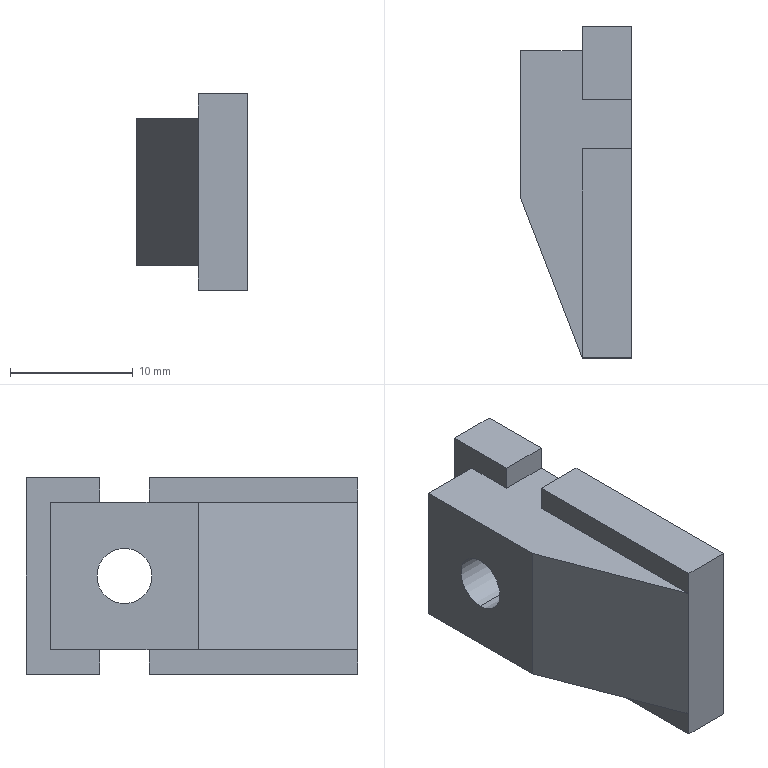Component | SolidWorks | ClampingBlock-2 | 1 solid | 24 faces | box 9 x 27 x 16 mm | volume 2480 mm3 | plane 20 | cylinder 4 | commonest cylinder face diameters 8 x2 4.5 x2
build123d program:
from build123d import *

# Parameters (mm, degrees)
BOSS_EXTRUDE1_DEPTH                             = 8
M4_HEX_SOCKET_HEAD_CAP_SCREW_CBORE2_D           = 4.5
M4_HEX_SOCKET_HEAD_CAP_SCREW_CBORE2_DEPTH       = 10.1
M4_HEX_SOCKET_HEAD_CAP_SCREW_CBORE2_CBORE_D     = 8
M4_HEX_SOCKET_HEAD_CAP_SCREW_CBORE2_CBORE_DEPTH = 4.4
M4_HEX_SOCKET_HEAD_CAP_SCREW_CBORE2_TIP         = 1.352
SKETCH4_W                                       = 5
SKETCH4_H                                       = 2
CUT_EXTRUDE1_DEPTH                              = 28.749
SKETCH5_W                                       = 2
SKETCH5_H                                       = 4
CUT_EXTRUDE2_DEPTH                              = 16


with BuildPart() as part:
    # Sketch1 → Boss-Extrude1 (new, symmetric)
    with BuildSketch(Plane.XY):
        Polygon((0, 0), (0, 27), (4, 27), (4, 25), (9, 25), (9, 13), (4, 0), align=None)
    extrude(amount=BOSS_EXTRUDE1_DEPTH, both=True)

    # M4 Hex Socket Head Cap Screw CBORE2
    with Locations(Plane(origin=(0, 19, 0), x_dir=(0, 0, -1), z_dir=(-1, 0, 0))):
        with Locations((0, 0)):
            CounterBoreHole(M4_HEX_SOCKET_HEAD_CAP_SCREW_CBORE2_D / 2, M4_HEX_SOCKET_HEAD_CAP_SCREW_CBORE2_CBORE_D / 2, M4_HEX_SOCKET_HEAD_CAP_SCREW_CBORE2_CBORE_DEPTH, depth=M4_HEX_SOCKET_HEAD_CAP_SCREW_CBORE2_DEPTH)
            with Locations((0, 0, -(M4_HEX_SOCKET_HEAD_CAP_SCREW_CBORE2_DEPTH + M4_HEX_SOCKET_HEAD_CAP_SCREW_CBORE2_TIP / 2))):  # 118° drill point
                Cone(0, M4_HEX_SOCKET_HEAD_CAP_SCREW_CBORE2_D / 2, M4_HEX_SOCKET_HEAD_CAP_SCREW_CBORE2_TIP, mode=Mode.SUBTRACT)

    # Sketch4 → Cut-Extrude1 (cut, through all)
    with BuildSketch(Plane(origin=(0, 25, 0), x_dir=(1, 0, 0), z_dir=(0, 1, 0))):
        with Locations((6.5, 7)):
            Rectangle(SKETCH4_W, SKETCH4_H)
        with Locations((6.5, -7)):
            Rectangle(SKETCH4_W, SKETCH4_H)
    extrude(amount=-CUT_EXTRUDE1_DEPTH, mode=Mode.SUBTRACT)

    # Sketch5 → Cut-Extrude2 (cut)
    with BuildSketch(Plane(origin=(4, 0, 0), x_dir=(0, 0, -1), z_dir=(1, 0, 0))):
        with Locations((-7, 19)):
            Rectangle(SKETCH5_W, SKETCH5_H)
        with Locations((7, 19)):
            Rectangle(SKETCH5_W, SKETCH5_H)
    extrude(amount=-CUT_EXTRUDE2_DEPTH, mode=Mode.SUBTRACT)


solid = part.part

# Placed as in the assembly
solid = solid.moved(Location((38.658, -220.962, 175.844), (-180, 0, 180)))
STEP:
#1=COLOUR_RGB('',0.7922,0.8196,0.9333);
#2=FILL_AREA_STYLE_COLOUR('',#1);
#3=FILL_AREA_STYLE('',(#2));
#4=SURFACE_STYLE_FILL_AREA(#3);
#5=SURFACE_SIDE_STYLE('',(#4));
#6=SURFACE_STYLE_USAGE(.BOTH.,#5);
#7=PRESENTATION_STYLE_ASSIGNMENT((#6));
#8=CARTESIAN_POINT('',(1.349,-7.951,7.08));
#9=VERTEX_POINT('',#8);
#10=CARTESIAN_POINT('',(1.349,-7.951,6.766));
#11=VERTEX_POINT('',#10);
#12=CARTESIAN_POINT('',(1.349,-7.951,6.923));
#13=DIRECTION('',(1.,-0.,0.));
#14=DIRECTION('',(0.,0.,-1.));
#15=AXIS2_PLACEMENT_3D('',#12,#13,#14);
#16=CIRCLE('',#15,0.1575);
#17=EDGE_CURVE('',#9,#11,#16,.T.);
#18=ORIENTED_EDGE('',*,*,#17,.F.);
#19=CARTESIAN_POINT('',(1.522,-7.951,7.08));
#20=VERTEX_POINT('',#19);
#21=CARTESIAN_POINT('',(1.522,-7.951,7.08));
#22=DIRECTION('',(1.,-0.,0.));
#23=VECTOR('',#22,39.37);
#24=LINE('',#21,#23);
#25=EDGE_CURVE('',#9,#20,#24,.T.);
#26=ORIENTED_EDGE('',*,*,#25,.T.);
#27=CARTESIAN_POINT('',(1.522,-7.951,6.766));
#28=VERTEX_POINT('',#27);
#29=CARTESIAN_POINT('',(1.522,-7.951,6.923));
#30=DIRECTION('',(1.,-0.,0.));
#31=DIRECTION('',(0.,0.,-1.));
#32=AXIS2_PLACEMENT_3D('',#29,#30,#31);
#33=CIRCLE('',#32,0.1575);
#34=EDGE_CURVE('',#20,#28,#33,.T.);
#35=ORIENTED_EDGE('',*,*,#34,.T.);
#36=CARTESIAN_POINT('',(1.522,-7.951,6.766));
#37=DIRECTION('',(1.,-0.,0.));
#38=VECTOR('',#37,39.37);
#39=LINE('',#36,#38);
#40=EDGE_CURVE('',#11,#28,#39,.T.);
#41=ORIENTED_EDGE('',*,*,#40,.F.);
#42=EDGE_LOOP('',(#18,#26,#35,#41));
#43=FACE_OUTER_BOUND('',#42,.T.);
#44=CARTESIAN_POINT('',(1.522,-7.951,6.923));
#45=DIRECTION('',(1.,-0.,0.));
#46=DIRECTION('',(0.,0.,-1.));
#47=AXIS2_PLACEMENT_3D('',#44,#45,#46);
#48=CYLINDRICAL_SURFACE('',#47,0.1575);
#49=ADVANCED_FACE('',(#43),#48,.F.);
#50=CARTESIAN_POINT('',(1.168,-7.951,7.012));
#51=VERTEX_POINT('',#50);
#52=CARTESIAN_POINT('',(1.168,-7.951,6.834));
#53=VERTEX_POINT('',#52);
#54=CARTESIAN_POINT('',(1.168,-7.951,6.923));
#55=DIRECTION('',(1.,-0.,0.));
#56=DIRECTION('',(0.,-1.,0.));
#57=AXIS2_PLACEMENT_3D('',#54,#55,#56);
#58=CIRCLE('',#57,0.08858);
#59=EDGE_CURVE('',#51,#53,#58,.T.);
#60=ORIENTED_EDGE('',*,*,#59,.F.);
#61=CARTESIAN_POINT('',(1.349,-7.951,7.012));
#62=VERTEX_POINT('',#61);
#63=CARTESIAN_POINT('',(1.522,-7.951,7.012));
#64=DIRECTION('',(1.,-0.,0.));
#65=VECTOR('',#64,39.37);
#66=LINE('',#63,#65);
#67=EDGE_CURVE('',#51,#62,#66,.T.);
#68=ORIENTED_EDGE('',*,*,#67,.T.);
#69=CARTESIAN_POINT('',(1.349,-7.951,6.834));
#70=VERTEX_POINT('',#69);
#71=CARTESIAN_POINT('',(1.349,-7.951,6.923));
#72=DIRECTION('',(1.,-0.,0.));
#73=DIRECTION('',(0.,0.,-1.));
#74=AXIS2_PLACEMENT_3D('',#71,#72,#73);
#75=CIRCLE('',#74,0.08858);
#76=EDGE_CURVE('',#62,#70,#75,.T.);
#77=ORIENTED_EDGE('',*,*,#76,.T.);
#78=CARTESIAN_POINT('',(1.522,-7.951,6.834));
#79=DIRECTION('',(1.,-0.,0.));
#80=VECTOR('',#79,39.37);
#81=LINE('',#78,#80);
#82=EDGE_CURVE('',#53,#70,#81,.T.);
#83=ORIENTED_EDGE('',*,*,#82,.F.);
#84=EDGE_LOOP('',(#60,#68,#77,#83));
#85=FACE_OUTER_BOUND('',#84,.T.);
#86=CARTESIAN_POINT('',(1.522,-7.951,6.923));
#87=DIRECTION('',(1.,-0.,0.));
#88=DIRECTION('',(0.,0.,-1.));
#89=AXIS2_PLACEMENT_3D('',#86,#87,#88);
#90=CYLINDRICAL_SURFACE('',#89,0.08858);
#91=ADVANCED_FACE('',(#85),#90,.F.);
#92=CARTESIAN_POINT('',(1.364,-7.873,7.159));
#93=VERTEX_POINT('',#92);
#94=CARTESIAN_POINT('',(1.364,-7.715,7.159));
#95=VERTEX_POINT('',#94);
#96=CARTESIAN_POINT('',(1.364,-8.699,7.159));
#97=DIRECTION('',(0.,1.,0.));
#98=VECTOR('',#97,39.37);
#99=LINE('',#96,#98);
#100=EDGE_CURVE('',#93,#95,#99,.T.);
#101=ORIENTED_EDGE('',*,*,#100,.F.);
#102=CARTESIAN_POINT('',(1.364,-7.873,7.238));
#103=VERTEX_POINT('',#102);
#104=CARTESIAN_POINT('',(1.364,-7.873,7.159));
#105=DIRECTION('',(0.,-0.,-1.));
#106=VECTOR('',#105,39.37);
#107=LINE('',#104,#106);
#108=EDGE_CURVE('',#103,#93,#107,.T.);
#109=ORIENTED_EDGE('',*,*,#108,.F.);
#110=CARTESIAN_POINT('',(1.364,-7.636,7.238));
#111=VERTEX_POINT('',#110);
#112=CARTESIAN_POINT('',(1.364,-7.636,7.238));
#113=DIRECTION('',(0.,1.,0.));
#114=VECTOR('',#113,39.37);
#115=LINE('',#112,#114);
#116=EDGE_CURVE('',#103,#111,#115,.T.);
#117=ORIENTED_EDGE('',*,*,#116,.T.);
#118=CARTESIAN_POINT('',(1.364,-7.636,6.608));
#119=VERTEX_POINT('',#118);
#120=CARTESIAN_POINT('',(1.364,-7.636,6.608));
#121=DIRECTION('',(-0.,0.,1.));
#122=VECTOR('',#121,39.37);
#123=LINE('',#120,#122);
#124=EDGE_CURVE('',#119,#111,#123,.T.);
#125=ORIENTED_EDGE('',*,*,#124,.F.);
#126=CARTESIAN_POINT('',(1.364,-7.873,6.608));
#127=VERTEX_POINT('',#126);
#128=CARTESIAN_POINT('',(1.364,-7.636,6.608));
#129=DIRECTION('',(0.,1.,0.));
#130=VECTOR('',#129,39.37);
#131=LINE('',#128,#130);
#132=EDGE_CURVE('',#127,#119,#131,.T.);
#133=ORIENTED_EDGE('',*,*,#132,.F.);
#134=CARTESIAN_POINT('',(1.364,-7.873,6.687));
#135=VERTEX_POINT('',#134);
#136=CARTESIAN_POINT('',(1.364,-7.873,6.608));
#137=DIRECTION('',(0.,-0.,-1.));
#138=VECTOR('',#137,39.37);
#139=LINE('',#136,#138);
#140=EDGE_CURVE('',#135,#127,#139,.T.);
#141=ORIENTED_EDGE('',*,*,#140,.F.);
#142=CARTESIAN_POINT('',(1.364,-7.715,6.687));
#143=VERTEX_POINT('',#142);
#144=CARTESIAN_POINT('',(1.364,-8.699,6.687));
#145=DIRECTION('',(0.,1.,0.));
#146=VECTOR('',#145,39.37);
#147=LINE('',#144,#146);
#148=EDGE_CURVE('',#135,#143,#147,.T.);
#149=ORIENTED_EDGE('',*,*,#148,.T.);
#150=CARTESIAN_POINT('',(1.364,-7.715,6.608));
#151=DIRECTION('',(-0.,0.,1.));
#152=VECTOR('',#151,39.37);
#153=LINE('',#150,#152);
#154=EDGE_CURVE('',#143,#95,#153,.T.);
#155=ORIENTED_EDGE('',*,*,#154,.T.);
#156=EDGE_LOOP('',(#101,#109,#117,#125,#133,#141,#149,#155));
#157=FACE_OUTER_BOUND('',#156,.T.);
#158=CARTESIAN_POINT('',(1.364,-7.636,6.608));
#159=DIRECTION('',(1.,-0.,0.));
#160=DIRECTION('',(0.,-0.,-1.));
#161=AXIS2_PLACEMENT_3D('',#158,#159,#160);
#162=PLANE('',#161);
#163=ADVANCED_FACE('',(#157),#162,.F.);
#164=CARTESIAN_POINT('',(1.522,-7.873,7.238));
#165=VERTEX_POINT('',#164);
#166=CARTESIAN_POINT('',(1.522,-7.873,7.238));
#167=DIRECTION('',(-1.,0.,-0.));
#168=VECTOR('',#167,39.37);
#169=LINE('',#166,#168);
#170=EDGE_CURVE('',#165,#103,#169,.T.);
#171=ORIENTED_EDGE('',*,*,#170,.F.);
#172=CARTESIAN_POINT('',(1.522,-7.636,7.238));
#173=VERTEX_POINT('',#172);
#174=CARTESIAN_POINT('',(1.522,-8.699,7.238));
#175=DIRECTION('',(-0.,-1.,-0.));
#176=VECTOR('',#175,39.37);
#177=LINE('',#174,#176);
#178=EDGE_CURVE('',#173,#165,#177,.T.);
#179=ORIENTED_EDGE('',*,*,#178,.F.);
#180=CARTESIAN_POINT('',(1.522,-7.636,7.238));
#181=DIRECTION('',(1.,-0.,0.));
#182=VECTOR('',#181,39.37);
#183=LINE('',#180,#182);
#184=EDGE_CURVE('',#111,#173,#183,.T.);
#185=ORIENTED_EDGE('',*,*,#184,.F.);
#186=ORIENTED_EDGE('',*,*,#116,.F.);
#187=EDGE_LOOP('',(#171,#179,#185,#186));
#188=FACE_OUTER_BOUND('',#187,.T.);
#189=CARTESIAN_POINT('',(1.522,-8.699,7.238));
#190=DIRECTION('',(-0.,0.,1.));
#191=DIRECTION('',(1.,-0.,0.));
#192=AXIS2_PLACEMENT_3D('',#189,#190,#191);
#193=PLANE('',#192);
#194=ADVANCED_FACE('',(#188),#193,.T.);
#195=CARTESIAN_POINT('',(1.364,-8.699,7.238));
#196=VERTEX_POINT('',#195);
#197=CARTESIAN_POINT('',(1.364,-8.03,7.238));
#198=VERTEX_POINT('',#197);
#199=CARTESIAN_POINT('',(1.364,-7.636,7.238));
#200=DIRECTION('',(0.,1.,0.));
#201=VECTOR('',#200,39.37);
#202=LINE('',#199,#201);
#203=EDGE_CURVE('',#196,#198,#202,.T.);
#204=ORIENTED_EDGE('',*,*,#203,.T.);
#205=CARTESIAN_POINT('',(1.364,-8.03,7.159));
#206=VERTEX_POINT('',#205);
#207=CARTESIAN_POINT('',(1.364,-8.03,7.159));
#208=DIRECTION('',(-0.,0.,1.));
#209=VECTOR('',#208,39.37);
#210=LINE('',#207,#209);
#211=EDGE_CURVE('',#206,#198,#210,.T.);
#212=ORIENTED_EDGE('',*,*,#211,.F.);
#213=CARTESIAN_POINT('',(1.364,-8.699,7.159));
#214=VERTEX_POINT('',#213);
#215=CARTESIAN_POINT('',(1.364,-8.699,7.159));
#216=DIRECTION('',(0.,1.,0.));
#217=VECTOR('',#216,39.37);
#218=LINE('',#215,#217);
#219=EDGE_CURVE('',#214,#206,#218,.T.);
#220=ORIENTED_EDGE('',*,*,#219,.F.);
#221=CARTESIAN_POINT('',(1.364,-8.699,7.238));
#222=DIRECTION('',(0.,-0.,-1.));
#223=VECTOR('',#222,39.37);
#224=LINE('',#221,#223);
#225=EDGE_CURVE('',#196,#214,#224,.T.);
#226=ORIENTED_EDGE('',*,*,#225,.F.);
#227=EDGE_LOOP('',(#204,#212,#220,#226));
#228=FACE_OUTER_BOUND('',#227,.T.);
#229=CARTESIAN_POINT('',(1.364,-7.636,6.608));
#230=DIRECTION('',(1.,-0.,0.));
#231=DIRECTION('',(0.,-0.,-1.));
#232=AXIS2_PLACEMENT_3D('',#229,#230,#231);
#233=PLANE('',#232);
#234=ADVANCED_FACE('',(#228),#233,.F.);
#235=CARTESIAN_POINT('',(1.522,-7.636,6.608));
#236=VERTEX_POINT('',#235);
#237=CARTESIAN_POINT('',(1.522,-7.873,6.608));
#238=VERTEX_POINT('',#237);
#239=CARTESIAN_POINT('',(1.522,-8.699,6.608));
#240=DIRECTION('',(-0.,-1.,-0.));
#241=VECTOR('',#240,39.37);
#242=LINE('',#239,#241);
#243=EDGE_CURVE('',#236,#238,#242,.T.);
#244=ORIENTED_EDGE('',*,*,#243,.T.);
#245=CARTESIAN_POINT('',(1.522,-7.873,6.608));
#246=DIRECTION('',(-1.,0.,-0.));
#247=VECTOR('',#246,39.37);
#248=LINE('',#245,#247);
#249=EDGE_CURVE('',#238,#127,#248,.T.);
#250=ORIENTED_EDGE('',*,*,#249,.T.);
#251=ORIENTED_EDGE('',*,*,#132,.T.);
#252=CARTESIAN_POINT('',(1.522,-7.636,6.608));
#253=DIRECTION('',(1.,-0.,0.));
#254=VECTOR('',#253,39.37);
#255=LINE('',#252,#254);
#256=EDGE_CURVE('',#119,#236,#255,.T.);
#257=ORIENTED_EDGE('',*,*,#256,.T.);
#258=EDGE_LOOP('',(#244,#250,#251,#257));
#259=FACE_OUTER_BOUND('',#258,.T.);
#260=CARTESIAN_POINT('',(1.522,-8.699,6.608));
#261=DIRECTION('',(-0.,0.,1.));
#262=DIRECTION('',(1.,-0.,0.));
#263=AXIS2_PLACEMENT_3D('',#260,#261,#262);
#264=PLANE('',#263);
#265=ADVANCED_FACE('',(#259),#264,.F.);
#266=CARTESIAN_POINT('',(1.522,-8.699,7.238));
#267=VERTEX_POINT('',#266);
#268=CARTESIAN_POINT('',(1.364,-8.699,7.238));
#269=DIRECTION('',(-1.,0.,-0.));
#270=VECTOR('',#269,39.37);
#271=LINE('',#268,#270);
#272=EDGE_CURVE('',#267,#196,#271,.T.);
#273=ORIENTED_EDGE('',*,*,#272,.T.);
#274=ORIENTED_EDGE('',*,*,#225,.T.);
#275=CARTESIAN_POINT('',(1.364,-8.699,6.687));
#276=VERTEX_POINT('',#275);
#277=CARTESIAN_POINT('',(1.364,-8.699,6.608));
#278=DIRECTION('',(-0.,0.,1.));
#279=VECTOR('',#278,39.37);
#280=LINE('',#277,#279);
#281=EDGE_CURVE('',#276,#214,#280,.T.);
#282=ORIENTED_EDGE('',*,*,#281,.F.);
#283=CARTESIAN_POINT('',(1.364,-8.699,6.608));
#284=VERTEX_POINT('',#283);
#285=CARTESIAN_POINT('',(1.364,-8.699,6.608));
#286=DIRECTION('',(-0.,0.,1.));
#287=VECTOR('',#286,39.37);
#288=LINE('',#285,#287);
#289=EDGE_CURVE('',#284,#276,#288,.T.);
#290=ORIENTED_EDGE('',*,*,#289,.F.);
#291=CARTESIAN_POINT('',(1.522,-8.699,6.608));
#292=VERTEX_POINT('',#291);
#293=CARTESIAN_POINT('',(1.364,-8.699,6.608));
#294=DIRECTION('',(-1.,0.,-0.));
#295=VECTOR('',#294,39.37);
#296=LINE('',#293,#295);
#297=EDGE_CURVE('',#292,#284,#296,.T.);
#298=ORIENTED_EDGE('',*,*,#297,.F.);
#299=CARTESIAN_POINT('',(1.522,-8.699,6.608));
#300=DIRECTION('',(-0.,0.,1.));
#301=VECTOR('',#300,39.37);
#302=LINE('',#299,#301);
#303=EDGE_CURVE('',#292,#267,#302,.T.);
#304=ORIENTED_EDGE('',*,*,#303,.T.);
#305=EDGE_LOOP('',(#273,#274,#282,#290,#298,#304));
#306=FACE_OUTER_BOUND('',#305,.T.);
#307=CARTESIAN_POINT('',(1.364,-8.699,6.608));
#308=DIRECTION('',(0.,1.,0.));
#309=DIRECTION('',(0.,-0.,-1.));
#310=AXIS2_PLACEMENT_3D('',#307,#308,#309);
#311=PLANE('',#310);
#312=ADVANCED_FACE('',(#306),#311,.F.);
#313=CARTESIAN_POINT('',(1.168,-8.187,6.687));
#314=VERTEX_POINT('',#313);
#315=CARTESIAN_POINT('',(1.168,-8.187,7.159));
#316=VERTEX_POINT('',#315);
#317=CARTESIAN_POINT('',(1.168,-8.187,6.608));
#318=DIRECTION('',(-0.,0.,1.));
#319=VECTOR('',#318,39.37);
#320=LINE('',#317,#319);
#321=EDGE_CURVE('',#314,#316,#320,.T.);
#322=ORIENTED_EDGE('',*,*,#321,.F.);
#323=CARTESIAN_POINT('',(1.168,-8.187,6.687));
#324=DIRECTION('',(0.359,-0.9333,0.));
#325=VECTOR('',#324,39.37);
#326=LINE('',#323,#325);
#327=EDGE_CURVE('',#314,#276,#326,.T.);
#328=ORIENTED_EDGE('',*,*,#327,.T.);
#329=ORIENTED_EDGE('',*,*,#281,.T.);
#330=CARTESIAN_POINT('',(1.168,-8.187,7.159));
#331=DIRECTION('',(-0.359,0.9333,-0.));
#332=VECTOR('',#331,39.37);
#333=LINE('',#330,#332);
#334=EDGE_CURVE('',#214,#316,#333,.T.);
#335=ORIENTED_EDGE('',*,*,#334,.T.);
#336=EDGE_LOOP('',(#322,#328,#329,#335));
#337=FACE_OUTER_BOUND('',#336,.T.);
#338=CARTESIAN_POINT('',(1.168,-8.187,6.608));
#339=DIRECTION('',(0.9333,0.359,0.));
#340=DIRECTION('',(0.359,-0.9333,0.));
#341=AXIS2_PLACEMENT_3D('',#338,#339,#340);
#342=PLANE('',#341);
#343=ADVANCED_FACE('',(#337),#342,.F.);
#344=CARTESIAN_POINT('',(1.168,-7.951,6.923));
#345=DIRECTION('',(1.,-0.,0.));
#346=DIRECTION('',(0.,-1.,0.));
#347=AXIS2_PLACEMENT_3D('',#344,#345,#346);
#348=CIRCLE('',#347,0.08858);
#349=EDGE_CURVE('',#53,#51,#348,.T.);
#350=ORIENTED_EDGE('',*,*,#349,.T.);
#351=ORIENTED_EDGE('',*,*,#59,.T.);
#352=EDGE_LOOP('',(#350,#351));
#353=FACE_BOUND('',#352,.T.);
#354=CARTESIAN_POINT('',(1.168,-7.715,6.687));
#355=VERTEX_POINT('',#354);
#356=CARTESIAN_POINT('',(1.168,-7.715,7.159));
#357=VERTEX_POINT('',#356);
#358=CARTESIAN_POINT('',(1.168,-7.715,6.608));
#359=DIRECTION('',(-0.,0.,1.));
#360=VECTOR('',#359,39.37);
#361=LINE('',#358,#360);
#362=EDGE_CURVE('',#355,#357,#361,.T.);
#363=ORIENTED_EDGE('',*,*,#362,.F.);
#364=CARTESIAN_POINT('',(1.168,-8.699,6.687));
#365=DIRECTION('',(0.,1.,0.));
#366=VECTOR('',#365,39.37);
#367=LINE('',#364,#366);
#368=EDGE_CURVE('',#314,#355,#367,.T.);
#369=ORIENTED_EDGE('',*,*,#368,.F.);
#370=ORIENTED_EDGE('',*,*,#321,.T.);
#371=CARTESIAN_POINT('',(1.168,-8.699,7.159));
#372=DIRECTION('',(0.,1.,0.));
#373=VECTOR('',#372,39.37);
#374=LINE('',#371,#373);
#375=EDGE_CURVE('',#316,#357,#374,.T.);
#376=ORIENTED_EDGE('',*,*,#375,.T.);
#377=EDGE_LOOP('',(#363,#369,#370,#376));
#378=FACE_OUTER_BOUND('',#377,.T.);
#379=CARTESIAN_POINT('',(1.168,-7.715,6.608));
#380=DIRECTION('',(1.,-0.,0.));
#381=DIRECTION('',(-0.,-1.,-0.));
#382=AXIS2_PLACEMENT_3D('',#379,#380,#381);
#383=PLANE('',#382);
#384=ADVANCED_FACE('',(#353,#378),#383,.F.);
#385=ORIENTED_EDGE('',*,*,#154,.F.);
#386=CARTESIAN_POINT('',(1.364,-7.715,6.687));
#387=DIRECTION('',(1.,-0.,0.));
#388=VECTOR('',#387,39.37);
#389=LINE('',#386,#388);
#390=EDGE_CURVE('',#355,#143,#389,.T.);
#391=ORIENTED_EDGE('',*,*,#390,.F.);
#392=ORIENTED_EDGE('',*,*,#362,.T.);
#393=CARTESIAN_POINT('',(1.364,-7.715,7.159));
#394=DIRECTION('',(-1.,0.,-0.));
#395=VECTOR('',#394,39.37);
#396=LINE('',#393,#395);
#397=EDGE_CURVE('',#95,#357,#396,.T.);
#398=ORIENTED_EDGE('',*,*,#397,.F.);
#399=EDGE_LOOP('',(#385,#391,#392,#398));
#400=FACE_OUTER_BOUND('',#399,.T.);
#401=CARTESIAN_POINT('',(1.364,-7.715,6.608));
#402=DIRECTION('',(-0.,-1.,-0.));
#403=DIRECTION('',(-0.,0.,1.));
#404=AXIS2_PLACEMENT_3D('',#401,#402,#403);
#405=PLANE('',#404);
#406=ADVANCED_FACE('',(#400),#405,.F.);
#407=CARTESIAN_POINT('',(1.364,-8.03,6.687));
#408=VERTEX_POINT('',#407);
#409=CARTESIAN_POINT('',(1.364,-8.699,6.687));
#410=DIRECTION('',(0.,1.,0.));
#411=VECTOR('',#410,39.37);
#412=LINE('',#409,#411);
#413=EDGE_CURVE('',#276,#408,#412,.T.);
#414=ORIENTED_EDGE('',*,*,#413,.T.);
#415=CARTESIAN_POINT('',(1.364,-8.03,6.608));
#416=VERTEX_POINT('',#415);
#417=CARTESIAN_POINT('',(1.364,-8.03,6.608));
#418=DIRECTION('',(-0.,0.,1.));
#419=VECTOR('',#418,39.37);
#420=LINE('',#417,#419);
#421=EDGE_CURVE('',#416,#408,#420,.T.);
#422=ORIENTED_EDGE('',*,*,#421,.F.);
#423=CARTESIAN_POINT('',(1.364,-7.636,6.608));
#424=DIRECTION('',(0.,1.,0.));
#425=VECTOR('',#424,39.37);
#426=LINE('',#423,#425);
#427=EDGE_CURVE('',#284,#416,#426,.T.);
#428=ORIENTED_EDGE('',*,*,#427,.F.);
#429=ORIENTED_EDGE('',*,*,#289,.T.);
#430=EDGE_LOOP('',(#414,#422,#428,#429));
#431=FACE_OUTER_BOUND('',#430,.T.);
#432=CARTESIAN_POINT('',(1.364,-7.636,6.608));
#433=DIRECTION('',(1.,-0.,0.));
#434=DIRECTION('',(0.,-0.,-1.));
#435=AXIS2_PLACEMENT_3D('',#432,#433,#434);
#436=PLANE('',#435);
#437=ADVANCED_FACE('',(#431),#436,.F.);
#438=ORIENTED_EDGE('',*,*,#184,.T.);
#439=CARTESIAN_POINT('',(1.522,-7.636,6.608));
#440=DIRECTION('',(-0.,0.,1.));
#441=VECTOR('',#440,39.37);
#442=LINE('',#439,#441);
#443=EDGE_CURVE('',#236,#173,#442,.T.);
#444=ORIENTED_EDGE('',*,*,#443,.F.);
#445=ORIENTED_EDGE('',*,*,#256,.F.);
#446=ORIENTED_EDGE('',*,*,#124,.T.);
#447=EDGE_LOOP('',(#438,#444,#445,#446));
#448=FACE_OUTER_BOUND('',#447,.T.);
#449=CARTESIAN_POINT('',(1.522,-7.636,6.608));
#450=DIRECTION('',(-0.,-1.,-0.));
#451=DIRECTION('',(-0.,0.,1.));
#452=AXIS2_PLACEMENT_3D('',#449,#450,#451);
#453=PLANE('',#452);
#454=ADVANCED_FACE('',(#448),#453,.F.);
#455=CARTESIAN_POINT('',(1.522,-7.951,6.923));
#456=DIRECTION('',(1.,-0.,0.));
#457=DIRECTION('',(0.,0.,-1.));
#458=AXIS2_PLACEMENT_3D('',#455,#456,#457);
#459=CIRCLE('',#458,0.1575);
#460=EDGE_CURVE('',#28,#20,#459,.T.);
#461=ORIENTED_EDGE('',*,*,#460,.F.);
#462=ORIENTED_EDGE('',*,*,#34,.F.);
#463=EDGE_LOOP('',(#461,#462));
#464=FACE_BOUND('',#463,.T.);
#465=ORIENTED_EDGE('',*,*,#178,.T.);
#466=CARTESIAN_POINT('',(1.522,-7.873,7.159));
#467=VERTEX_POINT('',#466);
#468=CARTESIAN_POINT('',(1.522,-7.873,6.608));
#469=DIRECTION('',(0.,-0.,-1.));
#470=VECTOR('',#469,39.37);
#471=LINE('',#468,#470);
#472=EDGE_CURVE('',#165,#467,#471,.T.);
#473=ORIENTED_EDGE('',*,*,#472,.T.);
#474=CARTESIAN_POINT('',(1.522,-8.03,7.159));
#475=VERTEX_POINT('',#474);
#476=CARTESIAN_POINT('',(1.522,-8.699,7.159));
#477=DIRECTION('',(-0.,-1.,0.));
#478=VECTOR('',#477,39.37);
#479=LINE('',#476,#478);
#480=EDGE_CURVE('',#467,#475,#479,.T.);
#481=ORIENTED_EDGE('',*,*,#480,.T.);
#482=CARTESIAN_POINT('',(1.522,-8.03,7.238));
#483=VERTEX_POINT('',#482);
#484=CARTESIAN_POINT('',(1.522,-8.03,6.608));
#485=DIRECTION('',(-0.,0.,1.));
#486=VECTOR('',#485,39.37);
#487=LINE('',#484,#486);
#488=EDGE_CURVE('',#475,#483,#487,.T.);
#489=ORIENTED_EDGE('',*,*,#488,.T.);
#490=CARTESIAN_POINT('',(1.522,-8.699,7.238));
#491=DIRECTION('',(-0.,-1.,-0.));
#492=VECTOR('',#491,39.37);
#493=LINE('',#490,#492);
#494=EDGE_CURVE('',#483,#267,#493,.T.);
#495=ORIENTED_EDGE('',*,*,#494,.T.);
#496=ORIENTED_EDGE('',*,*,#303,.F.);
#497=CARTESIAN_POINT('',(1.522,-8.03,6.608));
#498=VERTEX_POINT('',#497);
#499=CARTESIAN_POINT('',(1.522,-8.699,6.608));
#500=DIRECTION('',(-0.,-1.,-0.));
#501=VECTOR('',#500,39.37);
#502=LINE('',#499,#501);
#503=EDGE_CURVE('',#498,#292,#502,.T.);
#504=ORIENTED_EDGE('',*,*,#503,.F.);
#505=CARTESIAN_POINT('',(1.522,-8.03,6.687));
#506=VERTEX_POINT('',#505);
#507=CARTESIAN_POINT('',(1.522,-8.03,6.608));
#508=DIRECTION('',(-0.,0.,1.));
#509=VECTOR('',#508,39.37);
#510=LINE('',#507,#509);
#511=EDGE_CURVE('',#498,#506,#510,.T.);
#512=ORIENTED_EDGE('',*,*,#511,.T.);
#513=CARTESIAN_POINT('',(1.522,-7.873,6.687));
#514=VERTEX_POINT('',#513);
#515=CARTESIAN_POINT('',(1.522,-8.699,6.687));
#516=DIRECTION('',(0.,1.,0.));
#517=VECTOR('',#516,39.37);
#518=LINE('',#515,#517);
#519=EDGE_CURVE('',#506,#514,#518,.T.);
#520=ORIENTED_EDGE('',*,*,#519,.T.);
#521=CARTESIAN_POINT('',(1.522,-7.873,6.608));
#522=DIRECTION('',(0.,-0.,-1.));
#523=VECTOR('',#522,39.37);
#524=LINE('',#521,#523);
#525=EDGE_CURVE('',#514,#238,#524,.T.);
#526=ORIENTED_EDGE('',*,*,#525,.T.);
#527=ORIENTED_EDGE('',*,*,#243,.F.);
#528=ORIENTED_EDGE('',*,*,#443,.T.);
#529=EDGE_LOOP('',(#465,#473,#481,#489,#495,#496,#504,#512,#520,#526,#527,#528));
#530=FACE_OUTER_BOUND('',#529,.T.);
#531=CARTESIAN_POINT('',(1.522,-8.699,6.608));
#532=DIRECTION('',(-1.,0.,-0.));
#533=DIRECTION('',(-0.,0.,1.));
#534=AXIS2_PLACEMENT_3D('',#531,#532,#533);
#535=PLANE('',#534);
#536=ADVANCED_FACE('',(#464,#530),#535,.F.);
#537=ORIENTED_EDGE('',*,*,#427,.T.);
#538=CARTESIAN_POINT('',(1.522,-8.03,6.608));
#539=DIRECTION('',(1.,-0.,0.));
#540=VECTOR('',#539,39.37);
#541=LINE('',#538,#540);
#542=EDGE_CURVE('',#416,#498,#541,.T.);
#543=ORIENTED_EDGE('',*,*,#542,.T.);
#544=ORIENTED_EDGE('',*,*,#503,.T.);
#545=ORIENTED_EDGE('',*,*,#297,.T.);
#546=EDGE_LOOP('',(#537,#543,#544,#545));
#547=FACE_OUTER_BOUND('',#546,.T.);
#548=CARTESIAN_POINT('',(1.522,-8.699,6.608));
#549=DIRECTION('',(-0.,0.,1.));
#550=DIRECTION('',(1.,-0.,0.));
#551=AXIS2_PLACEMENT_3D('',#548,#549,#550);
#552=PLANE('',#551);
#553=ADVANCED_FACE('',(#547),#552,.F.);
#554=CARTESIAN_POINT('',(1.522,-8.03,7.238));
#555=DIRECTION('',(1.,-0.,0.));
#556=VECTOR('',#555,39.37);
#557=LINE('',#554,#556);
#558=EDGE_CURVE('',#198,#483,#557,.T.);
#559=ORIENTED_EDGE('',*,*,#558,.F.);
#560=ORIENTED_EDGE('',*,*,#203,.F.);
#561=ORIENTED_EDGE('',*,*,#272,.F.);
#562=ORIENTED_EDGE('',*,*,#494,.F.);
#563=EDGE_LOOP('',(#559,#560,#561,#562));
#564=FACE_OUTER_BOUND('',#563,.T.);
#565=CARTESIAN_POINT('',(1.522,-8.699,7.238));
#566=DIRECTION('',(-0.,0.,1.));
#567=DIRECTION('',(1.,-0.,0.));
#568=AXIS2_PLACEMENT_3D('',#565,#566,#567);
#569=PLANE('',#568);
#570=ADVANCED_FACE('',(#564),#569,.T.);
#571=ORIENTED_EDGE('',*,*,#67,.F.);
#572=ORIENTED_EDGE('',*,*,#349,.F.);
#573=ORIENTED_EDGE('',*,*,#82,.T.);
#574=CARTESIAN_POINT('',(1.349,-7.951,6.923));
#575=DIRECTION('',(1.,-0.,0.));
#576=DIRECTION('',(0.,0.,-1.));
#577=AXIS2_PLACEMENT_3D('',#574,#575,#576);
#578=CIRCLE('',#577,0.08858);
#579=EDGE_CURVE('',#70,#62,#578,.T.);
#580=ORIENTED_EDGE('',*,*,#579,.T.);
#581=EDGE_LOOP('',(#571,#572,#573,#580));
#582=FACE_OUTER_BOUND('',#581,.T.);
#583=CARTESIAN_POINT('',(1.522,-7.951,6.923));
#584=DIRECTION('',(1.,-0.,0.));
#585=DIRECTION('',(0.,0.,-1.));
#586=AXIS2_PLACEMENT_3D('',#583,#584,#585);
#587=CYLINDRICAL_SURFACE('',#586,0.08858);
#588=ADVANCED_FACE('',(#582),#587,.F.);
#589=ORIENTED_EDGE('',*,*,#579,.F.);
#590=ORIENTED_EDGE('',*,*,#76,.F.);
#591=EDGE_LOOP('',(#589,#590));
#592=FACE_BOUND('',#591,.T.);
#593=CARTESIAN_POINT('',(1.349,-7.951,6.923));
#594=DIRECTION('',(1.,-0.,0.));
#595=DIRECTION('',(0.,0.,-1.));
#596=AXIS2_PLACEMENT_3D('',#593,#594,#595);
#597=CIRCLE('',#596,0.1575);
#598=EDGE_CURVE('',#11,#9,#597,.T.);
#599=ORIENTED_EDGE('',*,*,#598,.T.);
#600=ORIENTED_EDGE('',*,*,#17,.T.);
#601=EDGE_LOOP('',(#599,#600));
#602=FACE_OUTER_BOUND('',#601,.T.);
#603=CARTESIAN_POINT('',(1.349,-7.863,6.923));
#604=DIRECTION('',(-1.,0.,-0.));
#605=DIRECTION('',(-0.,0.,1.));
#606=AXIS2_PLACEMENT_3D('',#603,#604,#605);
#607=PLANE('',#606);
#608=ADVANCED_FACE('',(#592,#602),#607,.F.);
#609=ORIENTED_EDGE('',*,*,#25,.F.);
#610=ORIENTED_EDGE('',*,*,#598,.F.);
#611=ORIENTED_EDGE('',*,*,#40,.T.);
#612=ORIENTED_EDGE('',*,*,#460,.T.);
#613=EDGE_LOOP('',(#609,#610,#611,#612));
#614=FACE_OUTER_BOUND('',#613,.T.);
#615=CARTESIAN_POINT('',(1.522,-7.951,6.923));
#616=DIRECTION('',(1.,-0.,0.));
#617=DIRECTION('',(0.,0.,-1.));
#618=AXIS2_PLACEMENT_3D('',#615,#616,#617);
#619=CYLINDRICAL_SURFACE('',#618,0.1575);
#620=ADVANCED_FACE('',(#614),#619,.F.);
#621=ORIENTED_EDGE('',*,*,#219,.T.);
#622=CARTESIAN_POINT('',(1.994,-8.03,7.159));
#623=DIRECTION('',(-1.,0.,-0.));
#624=VECTOR('',#623,39.37);
#625=LINE('',#622,#624);
#626=EDGE_CURVE('',#475,#206,#625,.T.);
#627=ORIENTED_EDGE('',*,*,#626,.F.);
#628=ORIENTED_EDGE('',*,*,#480,.F.);
#629=CARTESIAN_POINT('',(1.994,-7.873,7.159));
#630=DIRECTION('',(-1.,0.,-0.));
#631=VECTOR('',#630,39.37);
#632=LINE('',#629,#631);
#633=EDGE_CURVE('',#467,#93,#632,.T.);
#634=ORIENTED_EDGE('',*,*,#633,.T.);
#635=ORIENTED_EDGE('',*,*,#100,.T.);
#636=ORIENTED_EDGE('',*,*,#397,.T.);
#637=ORIENTED_EDGE('',*,*,#375,.F.);
#638=ORIENTED_EDGE('',*,*,#334,.F.);
#639=EDGE_LOOP('',(#621,#627,#628,#634,#635,#636,#637,#638));
#640=FACE_OUTER_BOUND('',#639,.T.);
#641=CARTESIAN_POINT('',(1.364,-8.699,7.159));
#642=DIRECTION('',(0.,-0.,-1.));
#643=DIRECTION('',(-1.,0.,-0.));
#644=AXIS2_PLACEMENT_3D('',#641,#642,#643);
#645=PLANE('',#644);
#646=ADVANCED_FACE('',(#640),#645,.F.);
#647=ORIENTED_EDGE('',*,*,#368,.T.);
#648=ORIENTED_EDGE('',*,*,#390,.T.);
#649=ORIENTED_EDGE('',*,*,#148,.F.);
#650=CARTESIAN_POINT('',(1.994,-7.873,6.687));
#651=DIRECTION('',(-1.,0.,-0.));
#652=VECTOR('',#651,39.37);
#653=LINE('',#650,#652);
#654=EDGE_CURVE('',#514,#135,#653,.T.);
#655=ORIENTED_EDGE('',*,*,#654,.F.);
#656=ORIENTED_EDGE('',*,*,#519,.F.);
#657=CARTESIAN_POINT('',(1.994,-8.03,6.687));
#658=DIRECTION('',(-1.,0.,-0.));
#659=VECTOR('',#658,39.37);
#660=LINE('',#657,#659);
#661=EDGE_CURVE('',#506,#408,#660,.T.);
#662=ORIENTED_EDGE('',*,*,#661,.T.);
#663=ORIENTED_EDGE('',*,*,#413,.F.);
#664=ORIENTED_EDGE('',*,*,#327,.F.);
#665=EDGE_LOOP('',(#647,#648,#649,#655,#656,#662,#663,#664));
#666=FACE_OUTER_BOUND('',#665,.T.);
#667=CARTESIAN_POINT('',(1.364,-8.699,6.687));
#668=DIRECTION('',(-0.,0.,1.));
#669=DIRECTION('',(1.,-0.,0.));
#670=AXIS2_PLACEMENT_3D('',#667,#668,#669);
#671=PLANE('',#670);
#672=ADVANCED_FACE('',(#666),#671,.F.);
#673=ORIENTED_EDGE('',*,*,#654,.T.);
#674=ORIENTED_EDGE('',*,*,#140,.T.);
#675=ORIENTED_EDGE('',*,*,#249,.F.);
#676=ORIENTED_EDGE('',*,*,#525,.F.);
#677=EDGE_LOOP('',(#673,#674,#675,#676));
#678=FACE_OUTER_BOUND('',#677,.T.);
#679=CARTESIAN_POINT('',(1.994,-7.873,6.608));
#680=DIRECTION('',(0.,1.,0.));
#681=DIRECTION('',(0.,-0.,-1.));
#682=AXIS2_PLACEMENT_3D('',#679,#680,#681);
#683=PLANE('',#682);
#684=ADVANCED_FACE('',(#678),#683,.F.);
#685=ORIENTED_EDGE('',*,*,#542,.F.);
#686=ORIENTED_EDGE('',*,*,#421,.T.);
#687=ORIENTED_EDGE('',*,*,#661,.F.);
#688=ORIENTED_EDGE('',*,*,#511,.F.);
#689=EDGE_LOOP('',(#685,#686,#687,#688));
#690=FACE_OUTER_BOUND('',#689,.T.);
#691=CARTESIAN_POINT('',(1.994,-8.03,6.608));
#692=DIRECTION('',(-0.,-1.,-0.));
#693=DIRECTION('',(-0.,0.,1.));
#694=AXIS2_PLACEMENT_3D('',#691,#692,#693);
#695=PLANE('',#694);
#696=ADVANCED_FACE('',(#690),#695,.F.);
#697=ORIENTED_EDGE('',*,*,#170,.T.);
#698=ORIENTED_EDGE('',*,*,#108,.T.);
#699=ORIENTED_EDGE('',*,*,#633,.F.);
#700=ORIENTED_EDGE('',*,*,#472,.F.);
#701=EDGE_LOOP('',(#697,#698,#699,#700));
#702=FACE_OUTER_BOUND('',#701,.T.);
#703=CARTESIAN_POINT('',(1.994,-7.873,7.159));
#704=DIRECTION('',(0.,1.,0.));
#705=DIRECTION('',(0.,-0.,-1.));
#706=AXIS2_PLACEMENT_3D('',#703,#704,#705);
#707=PLANE('',#706);
#708=ADVANCED_FACE('',(#702),#707,.F.);
#709=ORIENTED_EDGE('',*,*,#626,.T.);
#710=ORIENTED_EDGE('',*,*,#211,.T.);
#711=ORIENTED_EDGE('',*,*,#558,.T.);
#712=ORIENTED_EDGE('',*,*,#488,.F.);
#713=EDGE_LOOP('',(#709,#710,#711,#712));
#714=FACE_OUTER_BOUND('',#713,.T.);
#715=CARTESIAN_POINT('',(1.994,-8.03,7.159));
#716=DIRECTION('',(-0.,-1.,-0.));
#717=DIRECTION('',(-0.,0.,1.));
#718=AXIS2_PLACEMENT_3D('',#715,#716,#717);
#719=PLANE('',#718);
#720=ADVANCED_FACE('',(#714),#719,.F.);
#721=CLOSED_SHELL('',(#49,#91,#163,#194,#234,#265,#312,#343,#384,#406,#437,#454,#536,#553,#570,#588,#608,#620,#646,#672,#684,#696,#708,#720));
#722=MANIFOLD_SOLID_BREP('',#721);
#723=STYLED_ITEM('',(#7),#722);
#724=(LENGTH_UNIT()NAMED_UNIT(*)SI_UNIT($,.METRE.));
#725=LENGTH_MEASURE_WITH_UNIT(LENGTH_MEASURE(0.0254),#724);
#726=DIMENSIONAL_EXPONENTS(1.,0.,0.,0.,0.,0.,0.);
#727=(CONVERSION_BASED_UNIT('',#725)LENGTH_UNIT()NAMED_UNIT(#726));
#728=UNCERTAINTY_MEASURE_WITH_UNIT(LENGTH_MEASURE(0.00001),#727,'','');
#729=(NAMED_UNIT(*)PLANE_ANGLE_UNIT()SI_UNIT($,.RADIAN.));
#730=(NAMED_UNIT(*)SI_UNIT($,.STERADIAN.)SOLID_ANGLE_UNIT());
#731=(GEOMETRIC_REPRESENTATION_CONTEXT(3)GLOBAL_UNCERTAINTY_ASSIGNED_CONTEXT((#728))GLOBAL_UNIT_ASSIGNED_CONTEXT((#727,#729,#730))REPRESENTATION_CONTEXT('',''));
#732=MECHANICAL_DESIGN_GEOMETRIC_PRESENTATION_REPRESENTATION('',(#723),#731);
#733=PRESENTATION_LAYER_ASSIGNMENT('','',(#723));
#734=CARTESIAN_POINT('',(0.,0.,0.));
#735=DIRECTION('',(0.,0.,1.));
#736=DIRECTION('',(1.,0.,0.));
#737=AXIS2_PLACEMENT_3D('',#734,#735,#736);
#738=(LENGTH_UNIT()NAMED_UNIT(*)SI_UNIT($,.METRE.));
#739=LENGTH_MEASURE_WITH_UNIT(LENGTH_MEASURE(0.0254),#738);
#740=DIMENSIONAL_EXPONENTS(1.,0.,0.,0.,0.,0.,0.);
#741=(CONVERSION_BASED_UNIT('',#739)LENGTH_UNIT()NAMED_UNIT(#740));
#742=UNCERTAINTY_MEASURE_WITH_UNIT(LENGTH_MEASURE(0.00001),#741,'','');
#743=(NAMED_UNIT(*)PLANE_ANGLE_UNIT()SI_UNIT($,.RADIAN.));
#744=(NAMED_UNIT(*)SI_UNIT($,.STERADIAN.)SOLID_ANGLE_UNIT());
#745=(GEOMETRIC_REPRESENTATION_CONTEXT(3)GLOBAL_UNCERTAINTY_ASSIGNED_CONTEXT((#742))GLOBAL_UNIT_ASSIGNED_CONTEXT((#741,#743,#744))REPRESENTATION_CONTEXT('',''));
#746=ADVANCED_BREP_SHAPE_REPRESENTATION('',(#722,#737),#745);